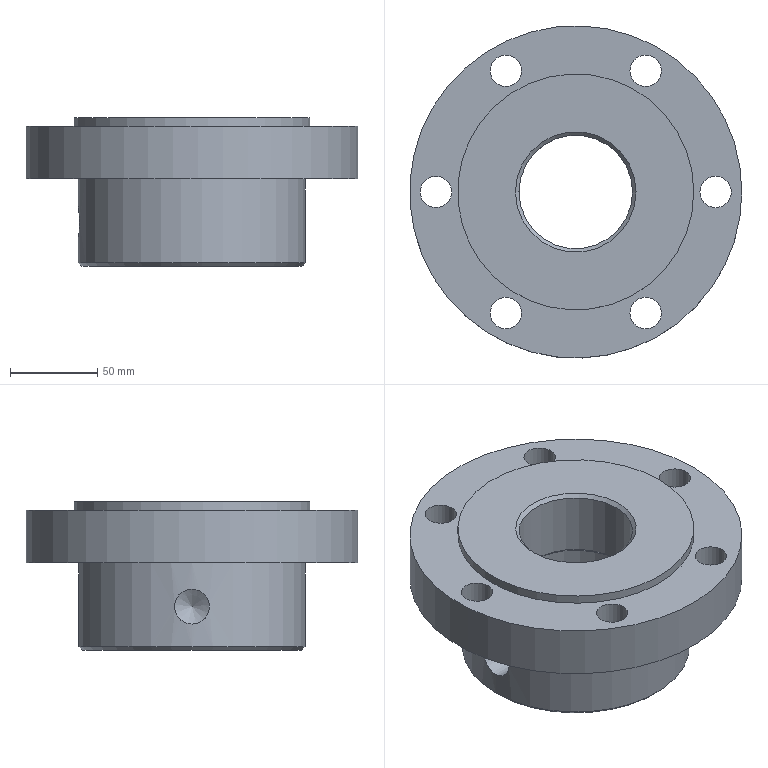Component | NX | CYLINDER_HEAD_BODY | 1 solid | 34 faces | volume 1182082 mm3 | cylinder 18 | plane 11 | cone 5 | commonest cylinder face diameters 18 x6 24 x6 130 x1 190 x1 135 x1 65 x1 75 x1 20 x1